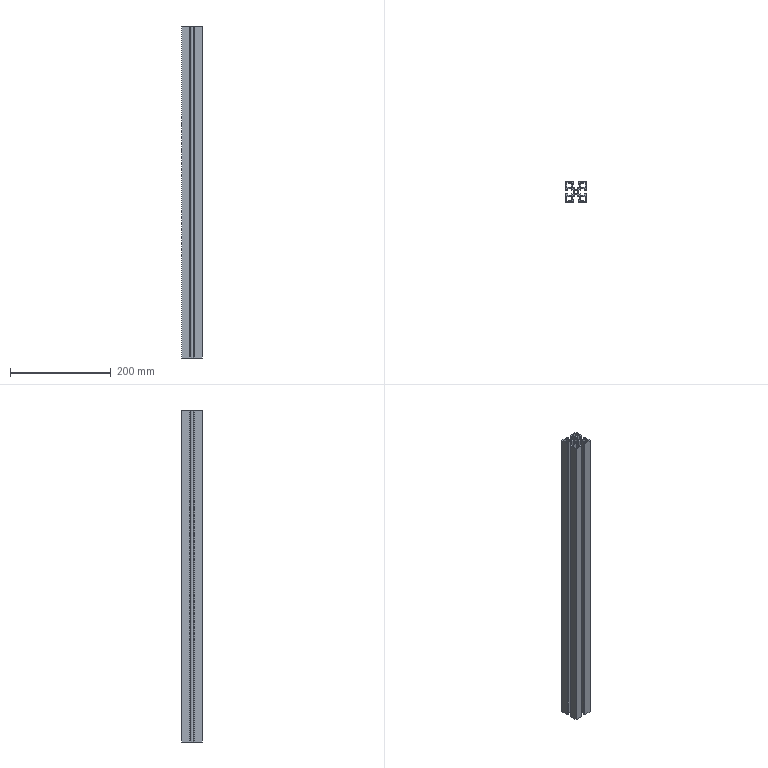Component | SolidWorks | AluminumProfile660-1 | 1 solid | 89 faces | box 40 x 40 x 660 mm | volume 382849 mm3 | plane 82 | cylinder 7 | commonest cylinder face diameters 10.5 x5 6.8 x2 | material 6061 Alloy
build123d program:
from build123d import *

# Parameters (mm, degrees)
SKETCH1_W                  = 40
SKETCH1_H                  = 40
EXTRUDE1_DEPTH             = 1640
CUT_EXTRUDE1_DEPTH         = 1641.975
SKETCH3_R                  = 3.4
CUT_EXTRUDE2_DEPTH         = 1641.975
CIRPATTERN1_COUNT          = 4
EXTRUDE2_DEPTH             = 1641.975
CIRPATTERN2_COUNT          = 4
SKETCH5_W                  = 9
SKETCH5_H                  = 9
EXTRUDE3_DEPTH             = 1641.975
CIRPATTERN3_COUNT          = 4
M8X1_25_TAPPED_HOLE3_D     = 6.8
M8X1_25_TAPPED_HOLE3_DEPTH = 19.75
M8X1_25_TAPPED_HOLE3_TIP   = 2.043
SKETCH9_W                  = 177.591
SKETCH9_H                  = 2021.808
CUT_EXTRUDE3_DEPTH         = 1641.975


with BuildPart() as part:
    # Sketch1 → Extrude1 (new body)
    with BuildSketch(Plane.XY):
        with Locations((20, 20)):
            Rectangle(SKETCH1_W, SKETCH1_H)
    extrude(amount=EXTRUDE1_DEPTH)

    # Sketch2 → Cut-Extrude1 (cut, through all)
    with BuildSketch(Plane.XY.offset(1640)):
        Polygon((16, 40), (16, 36), (13, 36), (13, 29), (27, 29), (27, 36), (24, 36), (24, 40), align=None)
    cut_extrude1 = extrude(amount=-CUT_EXTRUDE1_DEPTH, mode=Mode.SUBTRACT)

    # Sketch3 → Cut-Extrude2 (cut, through all)
    with BuildSketch(Plane.XY.offset(1640)):
        with Locations((20, 20)):
            Circle(SKETCH3_R)
    extrude(amount=-CUT_EXTRUDE2_DEPTH, mode=Mode.SUBTRACT)

    # CirPattern1: Cut-Extrude1 ×4 about axis
    cirpattern1_axis = Axis((20, 20, 0), (0, 0, 1))
    for i in range(1, CIRPATTERN1_COUNT):
        add(cut_extrude1.rotate(cirpattern1_axis, i * 360 / CIRPATTERN1_COUNT), mode=Mode.SUBTRACT)

    # Sketch4 → Extrude2 (cut, through all)
    with BuildSketch(Plane.XY.offset(1640)):
        with BuildLine():
            Line((15.75, 29), (16.457, 28.293))
            Line((16.457, 28.293), (14.806, 26.641))
            Line((14.806, 26.641), (17.082, 24.365))
            ThreePointArc((17.082, 24.365), (20, 25.25), (22.918, 24.365))
            Line((22.918, 24.365), (25.194, 26.641))
            Line((25.194, 26.641), (23.543, 28.293))
            Line((23.543, 28.293), (24.25, 29))
            Line((24.25, 29), (15.75, 29))
        make_face()
    extrude2 = extrude(amount=-EXTRUDE2_DEPTH, mode=Mode.SUBTRACT)

    # CirPattern2: Extrude2 ×4 about axis
    cirpattern2_axis = Axis((20, 20, 0), (0, 0, 1))
    for i in range(1, CIRPATTERN2_COUNT):
        add(extrude2.rotate(cirpattern2_axis, i * 360 / CIRPATTERN2_COUNT), mode=Mode.SUBTRACT)

    # Sketch5 → Extrude3 (cut, through all)
    with BuildSketch(Plane.XY.offset(1640)):
        with Locations((6.5, 33.5)):
            Rectangle(SKETCH5_W, SKETCH5_H)
    extrude3 = extrude(amount=-EXTRUDE3_DEPTH, mode=Mode.SUBTRACT)

    # CirPattern3: Extrude3 ×4 about axis
    cirpattern3_axis = Axis((20, 20, 0), (0, 0, 1))
    for i in range(1, CIRPATTERN3_COUNT):
        add(extrude3.rotate(cirpattern3_axis, i * 360 / CIRPATTERN3_COUNT), mode=Mode.SUBTRACT)

    # M8x1.25 Tapped Hole3
    with Locations(Plane(origin=(20, 20, 1640), x_dir=(1, 0, 0), z_dir=(0, 0, 1))):
        with Locations((0, 0)):
            Hole(M8X1_25_TAPPED_HOLE3_D / 2, depth=M8X1_25_TAPPED_HOLE3_DEPTH)
            with Locations((0, 0, -(M8X1_25_TAPPED_HOLE3_DEPTH + M8X1_25_TAPPED_HOLE3_TIP / 2))):  # 118° drill point
                Cone(0, M8X1_25_TAPPED_HOLE3_D / 2, M8X1_25_TAPPED_HOLE3_TIP, mode=Mode.SUBTRACT)

    # Sketch9 → Cut-Extrude3 (cut, through all)
    with BuildSketch(Plane.XZ):
        with Locations((13.869, 1670.904)):
            Rectangle(SKETCH9_W, SKETCH9_H)
    extrude(amount=-CUT_EXTRUDE3_DEPTH, mode=Mode.SUBTRACT)


solid = part.part

# Placed as in the assembly
solid = solid.moved(Location((-1288.352, -688.217, -16.285), (0, 0, 0)))